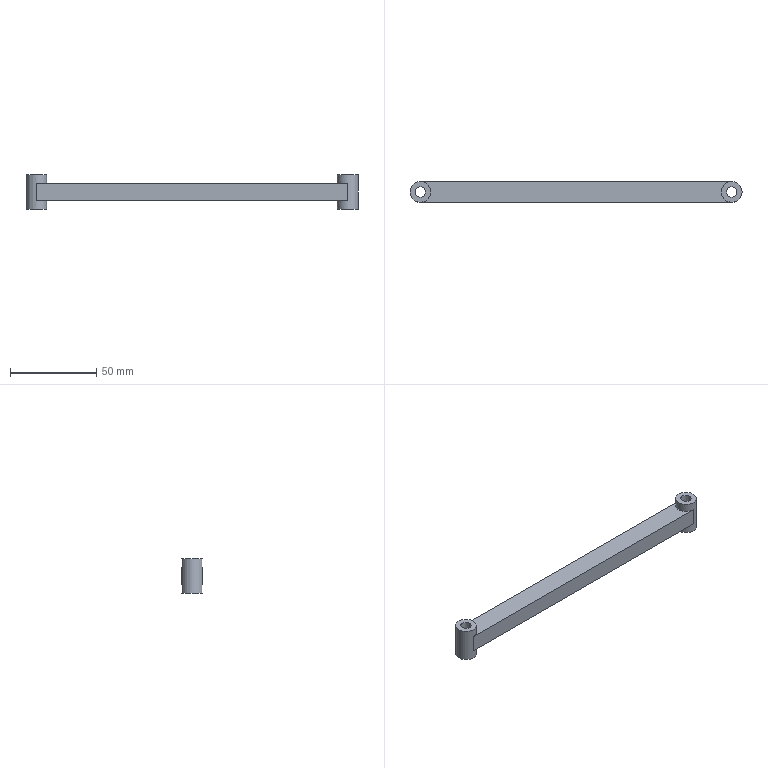Component | NX | CON_ROD2 | 1 solid | 12 faces | box 192 x 12 x 20 mm | volume 23862 mm3 | plane 8 | cylinder 4 | commonest cylinder face diameters 12 x2 6 x2
STEP:
#1=CARTESIAN_POINT('',(0.,0.,0.));
#2=DIRECTION('',(0.,0.,1.));
#3=DIRECTION('',(1.,0.,0.));
#4=AXIS2_PLACEMENT_3D('',#1,#2,#3);
#5=CARTESIAN_POINT('',(6.,65.,16.));
#6=VERTEX_POINT('',#5);
#7=CARTESIAN_POINT('',(-0.,65.,16.));
#8=DIRECTION('',(0.,0.,1.));
#9=DIRECTION('',(1.,0.,0.));
#10=AXIS2_PLACEMENT_3D('',#7,#8,#9);
#11=CIRCLE('',#10,6.);
#12=CARTESIAN_POINT('',(-0.,65.,36.));
#13=DIRECTION('',(0.,0.,-1.));
#14=DIRECTION('',(-1.,0.,0.));
#15=AXIS2_PLACEMENT_3D('',#12,#13,#14);
#16=CYLINDRICAL_SURFACE('',#15,6.);
#17=CARTESIAN_POINT('',(9.425,20.));
#18=DIRECTION('',(-1.,0.));
#19=VECTOR('',#18,1.);
#20=LINE('',#17,#19);
#21=(GEOMETRIC_REPRESENTATION_CONTEXT(2)PARAMETRIC_REPRESENTATION_CONTEXT()REPRESENTATION_CONTEXT('',''));
#22=DEFINITIONAL_REPRESENTATION('',(#20),#21);
#23=PCURVE('',#16,#22);
#24=CARTESIAN_POINT('',(-0.,65.,16.));
#25=DIRECTION('',(0.,0.,1.));
#26=DIRECTION('',(1.,0.,0.));
#27=AXIS2_PLACEMENT_3D('',#24,#25,#26);
#28=PLANE('',#27);
#29=CARTESIAN_POINT('',(0.,0.));
#30=DIRECTION('',(1.,0.));
#31=AXIS2_PLACEMENT_2D('',#29,#30);
#32=CIRCLE('',#31,6.);
#33=(GEOMETRIC_REPRESENTATION_CONTEXT(2)PARAMETRIC_REPRESENTATION_CONTEXT()REPRESENTATION_CONTEXT('',''));
#34=DEFINITIONAL_REPRESENTATION('',(#32),#33);
#35=PCURVE('',#28,#34);
#36=SURFACE_CURVE('',#11,(#23,#35),.PCURVE_S1.);
#37=EDGE_CURVE('',#6,#6,#36,.T.);
#38=ORIENTED_EDGE('',*,*,#37,.T.);
#39=CARTESIAN_POINT('',(6.,65.,21.));
#40=VERTEX_POINT('',#39);
#41=CARTESIAN_POINT('',(6.,65.,21.));
#42=CARTESIAN_POINT('',(6.,65.,16.));
#43=B_SPLINE_CURVE_WITH_KNOTS('',1,(#41,#42),.UNSPECIFIED.,.F.,.F.,(2,2),(15.,20.),.PIECEWISE_BEZIER_KNOTS.);
#44=CARTESIAN_POINT('',(3.142,0.));
#45=DIRECTION('',(0.,1.));
#46=VECTOR('',#45,1.);
#47=LINE('',#44,#46);
#48=(GEOMETRIC_REPRESENTATION_CONTEXT(2)PARAMETRIC_REPRESENTATION_CONTEXT()REPRESENTATION_CONTEXT('',''));
#49=DEFINITIONAL_REPRESENTATION('',(#47),#48);
#50=PCURVE('',#16,#49);
#51=CARTESIAN_POINT('',(9.425,0.));
#52=DIRECTION('',(0.,1.));
#53=VECTOR('',#52,1.);
#54=LINE('',#51,#53);
#55=(GEOMETRIC_REPRESENTATION_CONTEXT(2)PARAMETRIC_REPRESENTATION_CONTEXT()REPRESENTATION_CONTEXT('',''));
#56=DEFINITIONAL_REPRESENTATION('',(#54),#55);
#57=PCURVE('',#16,#56);
#58=SEAM_CURVE('',#43,(#50,#57),.PCURVE_S1.);
#59=EDGE_CURVE('',#40,#6,#58,.T.);
#60=ORIENTED_EDGE('',*,*,#59,.F.);
#61=CARTESIAN_POINT('',(-0.,59.,21.));
#62=VERTEX_POINT('',#61);
#63=CARTESIAN_POINT('',(-0.,65.,21.));
#64=DIRECTION('',(0.,0.,-1.));
#65=DIRECTION('',(-1.,0.,0.));
#66=AXIS2_PLACEMENT_3D('',#63,#64,#65);
#67=CIRCLE('',#66,6.);
#68=CARTESIAN_POINT('',(0.,15.));
#69=DIRECTION('',(1.,0.));
#70=VECTOR('',#69,1.);
#71=LINE('',#68,#70);
#72=(GEOMETRIC_REPRESENTATION_CONTEXT(2)PARAMETRIC_REPRESENTATION_CONTEXT()REPRESENTATION_CONTEXT('',''));
#73=DEFINITIONAL_REPRESENTATION('',(#71),#72);
#74=PCURVE('',#16,#73);
#75=CARTESIAN_POINT('',(-0.,65.,21.));
#76=DIRECTION('',(0.,0.,-1.));
#77=DIRECTION('',(1.,0.,0.));
#78=AXIS2_PLACEMENT_3D('',#75,#76,#77);
#79=PLANE('',#78);
#80=CARTESIAN_POINT('',(0.,0.));
#81=DIRECTION('',(-1.,0.));
#82=AXIS2_PLACEMENT_2D('',#80,#81);
#83=CIRCLE('',#82,6.);
#84=(GEOMETRIC_REPRESENTATION_CONTEXT(2)PARAMETRIC_REPRESENTATION_CONTEXT()REPRESENTATION_CONTEXT('',''));
#85=DEFINITIONAL_REPRESENTATION('',(#83),#84);
#86=PCURVE('',#79,#85);
#87=SURFACE_CURVE('',#67,(#74,#86),.PCURVE_S1.);
#88=EDGE_CURVE('',#40,#62,#87,.T.);
#89=ORIENTED_EDGE('',*,*,#88,.T.);
#90=CARTESIAN_POINT('',(-0.,59.,31.));
#91=VERTEX_POINT('',#90);
#92=CARTESIAN_POINT('',(-0.,59.,21.));
#93=DIRECTION('',(0.,0.,1.));
#94=VECTOR('',#93,1.);
#95=LINE('',#92,#94);
#96=CARTESIAN_POINT('',(4.712,15.));
#97=DIRECTION('',(0.,-1.));
#98=VECTOR('',#97,1.);
#99=LINE('',#96,#98);
#100=(GEOMETRIC_REPRESENTATION_CONTEXT(2)PARAMETRIC_REPRESENTATION_CONTEXT()REPRESENTATION_CONTEXT('',''));
#101=DEFINITIONAL_REPRESENTATION('',(#99),#100);
#102=PCURVE('',#16,#101);
#103=CARTESIAN_POINT('',(-0.,59.,21.));
#104=DIRECTION('',(0.,-1.,0.));
#105=DIRECTION('',(0.,0.,-1.));
#106=AXIS2_PLACEMENT_3D('',#103,#104,#105);
#107=PLANE('',#106);
#108=CARTESIAN_POINT('',(0.,0.));
#109=DIRECTION('',(-1.,0.));
#110=VECTOR('',#109,1.);
#111=LINE('',#108,#110);
#112=(GEOMETRIC_REPRESENTATION_CONTEXT(2)PARAMETRIC_REPRESENTATION_CONTEXT()REPRESENTATION_CONTEXT('',''));
#113=DEFINITIONAL_REPRESENTATION('',(#111),#112);
#114=PCURVE('',#107,#113);
#115=SURFACE_CURVE('',#95,(#102,#114),.PCURVE_S1.);
#116=EDGE_CURVE('',#62,#91,#115,.T.);
#117=ORIENTED_EDGE('',*,*,#116,.T.);
#118=CARTESIAN_POINT('',(6.,65.,31.));
#119=VERTEX_POINT('',#118);
#120=CARTESIAN_POINT('',(-0.,65.,31.));
#121=DIRECTION('',(0.,0.,1.));
#122=DIRECTION('',(-1.,0.,0.));
#123=AXIS2_PLACEMENT_3D('',#120,#121,#122);
#124=CIRCLE('',#123,6.);
#125=CARTESIAN_POINT('',(6.283,5.));
#126=DIRECTION('',(-1.,0.));
#127=VECTOR('',#126,1.);
#128=LINE('',#125,#127);
#129=(GEOMETRIC_REPRESENTATION_CONTEXT(2)PARAMETRIC_REPRESENTATION_CONTEXT()REPRESENTATION_CONTEXT('',''));
#130=DEFINITIONAL_REPRESENTATION('',(#128),#129);
#131=PCURVE('',#16,#130);
#132=CARTESIAN_POINT('',(-0.,65.,31.));
#133=DIRECTION('',(0.,0.,-1.));
#134=DIRECTION('',(1.,0.,0.));
#135=AXIS2_PLACEMENT_3D('',#132,#133,#134);
#136=PLANE('',#135);
#137=CARTESIAN_POINT('',(-6.,0.));
#138=CARTESIAN_POINT('',(-6.,10.392));
#139=CARTESIAN_POINT('',(3.,5.196));
#140=CARTESIAN_POINT('',(12.,0.));
#141=CARTESIAN_POINT('',(3.,-5.196));
#142=CARTESIAN_POINT('',(-6.,-10.392));
#143=CARTESIAN_POINT('',(-6.,0.));
#144=(BOUNDED_CURVE()B_SPLINE_CURVE(2,(#137,#138,#139,#140,#141,#142,#143),.UNSPECIFIED.,.T.,.F.)B_SPLINE_CURVE_WITH_KNOTS((1,2,2,2,2,1),(-2.094,0.,2.094,4.189,6.283,8.378),.UNSPECIFIED.)CURVE()GEOMETRIC_REPRESENTATION_ITEM()RATIONAL_B_SPLINE_CURVE((1.,0.5,1.,0.5,1.,0.5,1.))REPRESENTATION_ITEM(''));
#145=(GEOMETRIC_REPRESENTATION_CONTEXT(2)PARAMETRIC_REPRESENTATION_CONTEXT()REPRESENTATION_CONTEXT('',''));
#146=DEFINITIONAL_REPRESENTATION('',(#144),#145);
#147=PCURVE('',#136,#146);
#148=SURFACE_CURVE('',#124,(#131,#147),.PCURVE_S1.);
#149=EDGE_CURVE('',#91,#119,#148,.T.);
#150=ORIENTED_EDGE('',*,*,#149,.T.);
#151=CARTESIAN_POINT('',(6.,65.,36.));
#152=VERTEX_POINT('',#151);
#153=CARTESIAN_POINT('',(6.,65.,36.));
#154=CARTESIAN_POINT('',(6.,65.,31.));
#155=B_SPLINE_CURVE_WITH_KNOTS('',1,(#153,#154),.UNSPECIFIED.,.F.,.F.,(2,2),(0.,5.),.PIECEWISE_BEZIER_KNOTS.);
#156=CARTESIAN_POINT('',(3.142,0.));
#157=DIRECTION('',(0.,1.));
#158=VECTOR('',#157,1.);
#159=LINE('',#156,#158);
#160=(GEOMETRIC_REPRESENTATION_CONTEXT(2)PARAMETRIC_REPRESENTATION_CONTEXT()REPRESENTATION_CONTEXT('',''));
#161=DEFINITIONAL_REPRESENTATION('',(#159),#160);
#162=PCURVE('',#16,#161);
#163=CARTESIAN_POINT('',(9.425,0.));
#164=DIRECTION('',(0.,1.));
#165=VECTOR('',#164,1.);
#166=LINE('',#163,#165);
#167=(GEOMETRIC_REPRESENTATION_CONTEXT(2)PARAMETRIC_REPRESENTATION_CONTEXT()REPRESENTATION_CONTEXT('',''));
#168=DEFINITIONAL_REPRESENTATION('',(#166),#167);
#169=PCURVE('',#16,#168);
#170=SEAM_CURVE('',#155,(#162,#169),.PCURVE_S1.);
#171=EDGE_CURVE('',#152,#119,#170,.T.);
#172=ORIENTED_EDGE('',*,*,#171,.F.);
#173=CARTESIAN_POINT('',(-0.,65.,36.));
#174=DIRECTION('',(0.,0.,1.));
#175=DIRECTION('',(1.,0.,0.));
#176=AXIS2_PLACEMENT_3D('',#173,#174,#175);
#177=CIRCLE('',#176,6.);
#178=CARTESIAN_POINT('',(9.425,0.));
#179=DIRECTION('',(-1.,0.));
#180=VECTOR('',#179,1.);
#181=LINE('',#178,#180);
#182=(GEOMETRIC_REPRESENTATION_CONTEXT(2)PARAMETRIC_REPRESENTATION_CONTEXT()REPRESENTATION_CONTEXT('',''));
#183=DEFINITIONAL_REPRESENTATION('',(#181),#182);
#184=PCURVE('',#16,#183);
#185=CARTESIAN_POINT('',(-0.,65.,36.));
#186=DIRECTION('',(0.,0.,1.));
#187=DIRECTION('',(1.,0.,0.));
#188=AXIS2_PLACEMENT_3D('',#185,#186,#187);
#189=PLANE('',#188);
#190=CARTESIAN_POINT('',(0.,0.));
#191=DIRECTION('',(1.,0.));
#192=AXIS2_PLACEMENT_2D('',#190,#191);
#193=CIRCLE('',#192,6.);
#194=(GEOMETRIC_REPRESENTATION_CONTEXT(2)PARAMETRIC_REPRESENTATION_CONTEXT()REPRESENTATION_CONTEXT('',''));
#195=DEFINITIONAL_REPRESENTATION('',(#193),#194);
#196=PCURVE('',#189,#195);
#197=SURFACE_CURVE('',#177,(#184,#196),.PCURVE_S1.);
#198=EDGE_CURVE('',#152,#152,#197,.T.);
#199=ORIENTED_EDGE('',*,*,#198,.F.);
#200=ORIENTED_EDGE('',*,*,#171,.T.);
#201=CARTESIAN_POINT('',(-0.,71.,31.));
#202=VERTEX_POINT('',#201);
#203=CARTESIAN_POINT('',(-0.,65.,31.));
#204=DIRECTION('',(0.,0.,1.));
#205=DIRECTION('',(-1.,0.,0.));
#206=AXIS2_PLACEMENT_3D('',#203,#204,#205);
#207=CIRCLE('',#206,6.);
#208=CARTESIAN_POINT('',(12.566,5.));
#209=DIRECTION('',(-1.,0.));
#210=VECTOR('',#209,1.);
#211=LINE('',#208,#210);
#212=(GEOMETRIC_REPRESENTATION_CONTEXT(2)PARAMETRIC_REPRESENTATION_CONTEXT()REPRESENTATION_CONTEXT('',''));
#213=DEFINITIONAL_REPRESENTATION('',(#211),#212);
#214=PCURVE('',#16,#213);
#215=CARTESIAN_POINT('',(-6.,0.));
#216=CARTESIAN_POINT('',(-6.,10.392));
#217=CARTESIAN_POINT('',(3.,5.196));
#218=CARTESIAN_POINT('',(12.,0.));
#219=CARTESIAN_POINT('',(3.,-5.196));
#220=CARTESIAN_POINT('',(-6.,-10.392));
#221=CARTESIAN_POINT('',(-6.,0.));
#222=(BOUNDED_CURVE()B_SPLINE_CURVE(2,(#215,#216,#217,#218,#219,#220,#221),.UNSPECIFIED.,.T.,.F.)B_SPLINE_CURVE_WITH_KNOTS((1,2,2,2,2,1),(-2.094,0.,2.094,4.189,6.283,8.378),.UNSPECIFIED.)CURVE()GEOMETRIC_REPRESENTATION_ITEM()RATIONAL_B_SPLINE_CURVE((1.,0.5,1.,0.5,1.,0.5,1.))REPRESENTATION_ITEM(''));
#223=(GEOMETRIC_REPRESENTATION_CONTEXT(2)PARAMETRIC_REPRESENTATION_CONTEXT()REPRESENTATION_CONTEXT('',''));
#224=DEFINITIONAL_REPRESENTATION('',(#222),#223);
#225=PCURVE('',#136,#224);
#226=SURFACE_CURVE('',#207,(#214,#225),.PCURVE_S1.);
#227=EDGE_CURVE('',#119,#202,#226,.T.);
#228=ORIENTED_EDGE('',*,*,#227,.T.);
#229=CARTESIAN_POINT('',(-0.,71.,21.));
#230=VERTEX_POINT('',#229);
#231=CARTESIAN_POINT('',(-0.,71.,21.));
#232=DIRECTION('',(0.,0.,1.));
#233=VECTOR('',#232,1.);
#234=LINE('',#231,#233);
#235=CARTESIAN_POINT('',(7.854,15.));
#236=DIRECTION('',(0.,-1.));
#237=VECTOR('',#236,1.);
#238=LINE('',#235,#237);
#239=(GEOMETRIC_REPRESENTATION_CONTEXT(2)PARAMETRIC_REPRESENTATION_CONTEXT()REPRESENTATION_CONTEXT('',''));
#240=DEFINITIONAL_REPRESENTATION('',(#238),#239);
#241=PCURVE('',#16,#240);
#242=CARTESIAN_POINT('',(-0.,71.,21.));
#243=DIRECTION('',(0.,-1.,0.));
#244=DIRECTION('',(0.,0.,-1.));
#245=AXIS2_PLACEMENT_3D('',#242,#243,#244);
#246=PLANE('',#245);
#247=CARTESIAN_POINT('',(0.,0.));
#248=DIRECTION('',(-1.,0.));
#249=VECTOR('',#248,1.);
#250=LINE('',#247,#249);
#251=(GEOMETRIC_REPRESENTATION_CONTEXT(2)PARAMETRIC_REPRESENTATION_CONTEXT()REPRESENTATION_CONTEXT('',''));
#252=DEFINITIONAL_REPRESENTATION('',(#250),#251);
#253=PCURVE('',#246,#252);
#254=SURFACE_CURVE('',#234,(#241,#253),.PCURVE_S1.);
#255=EDGE_CURVE('',#230,#202,#254,.T.);
#256=ORIENTED_EDGE('',*,*,#255,.F.);
#257=CARTESIAN_POINT('',(-0.,65.,21.));
#258=DIRECTION('',(0.,0.,-1.));
#259=DIRECTION('',(-1.,0.,0.));
#260=AXIS2_PLACEMENT_3D('',#257,#258,#259);
#261=CIRCLE('',#260,6.);
#262=CARTESIAN_POINT('',(6.283,15.));
#263=DIRECTION('',(1.,0.));
#264=VECTOR('',#263,1.);
#265=LINE('',#262,#264);
#266=(GEOMETRIC_REPRESENTATION_CONTEXT(2)PARAMETRIC_REPRESENTATION_CONTEXT()REPRESENTATION_CONTEXT('',''));
#267=DEFINITIONAL_REPRESENTATION('',(#265),#266);
#268=PCURVE('',#16,#267);
#269=CARTESIAN_POINT('',(0.,0.));
#270=DIRECTION('',(-1.,0.));
#271=AXIS2_PLACEMENT_2D('',#269,#270);
#272=CIRCLE('',#271,6.);
#273=(GEOMETRIC_REPRESENTATION_CONTEXT(2)PARAMETRIC_REPRESENTATION_CONTEXT()REPRESENTATION_CONTEXT('',''));
#274=DEFINITIONAL_REPRESENTATION('',(#272),#273);
#275=PCURVE('',#79,#274);
#276=SURFACE_CURVE('',#261,(#268,#275),.PCURVE_S1.);
#277=EDGE_CURVE('',#230,#40,#276,.T.);
#278=ORIENTED_EDGE('',*,*,#277,.T.);
#279=ORIENTED_EDGE('',*,*,#59,.T.);
#280=EDGE_LOOP('',(#38,#60,#89,#117,#150,#172,#199,#200,#228,#256,#278,#279));
#281=FACE_BOUND('',#280,.T.);
#282=ADVANCED_FACE('',(#281),#16,.T.);
#283=CARTESIAN_POINT('',(-3.,65.,36.));
#284=VERTEX_POINT('',#283);
#285=CARTESIAN_POINT('',(-0.,65.,36.));
#286=DIRECTION('',(0.,0.,-1.));
#287=DIRECTION('',(-1.,0.,0.));
#288=AXIS2_PLACEMENT_3D('',#285,#286,#287);
#289=CIRCLE('',#288,3.);
#290=CARTESIAN_POINT('',(-3.,0.));
#291=CARTESIAN_POINT('',(-3.,5.196));
#292=CARTESIAN_POINT('',(1.5,2.598));
#293=CARTESIAN_POINT('',(6.,0.));
#294=CARTESIAN_POINT('',(1.5,-2.598));
#295=CARTESIAN_POINT('',(-3.,-5.196));
#296=CARTESIAN_POINT('',(-3.,0.));
#297=(BOUNDED_CURVE()B_SPLINE_CURVE(2,(#290,#291,#292,#293,#294,#295,#296),.UNSPECIFIED.,.T.,.F.)B_SPLINE_CURVE_WITH_KNOTS((1,2,2,2,2,1),(-2.094,0.,2.094,4.189,6.283,8.378),.UNSPECIFIED.)CURVE()GEOMETRIC_REPRESENTATION_ITEM()RATIONAL_B_SPLINE_CURVE((1.,0.5,1.,0.5,1.,0.5,1.))REPRESENTATION_ITEM(''));
#298=(GEOMETRIC_REPRESENTATION_CONTEXT(2)PARAMETRIC_REPRESENTATION_CONTEXT()REPRESENTATION_CONTEXT('',''));
#299=DEFINITIONAL_REPRESENTATION('',(#297),#298);
#300=PCURVE('',#189,#299);
#301=CARTESIAN_POINT('',(-0.,65.,36.));
#302=DIRECTION('',(0.,0.,-1.));
#303=DIRECTION('',(-1.,0.,0.));
#304=AXIS2_PLACEMENT_3D('',#301,#302,#303);
#305=CYLINDRICAL_SURFACE('',#304,3.);
#306=CARTESIAN_POINT('',(0.,0.));
#307=DIRECTION('',(1.,0.));
#308=VECTOR('',#307,1.);
#309=LINE('',#306,#308);
#310=(GEOMETRIC_REPRESENTATION_CONTEXT(2)PARAMETRIC_REPRESENTATION_CONTEXT()REPRESENTATION_CONTEXT('',''));
#311=DEFINITIONAL_REPRESENTATION('',(#309),#310);
#312=PCURVE('',#305,#311);
#313=SURFACE_CURVE('',#289,(#300,#312),.PCURVE_S1.);
#314=EDGE_CURVE('',#284,#284,#313,.T.);
#315=ORIENTED_EDGE('',*,*,#314,.T.);
#316=EDGE_LOOP('',(#315));
#317=FACE_BOUND('',#316,.T.);
#318=ORIENTED_EDGE('',*,*,#198,.T.);
#319=EDGE_LOOP('',(#318));
#320=FACE_BOUND('',#319,.T.);
#321=ADVANCED_FACE('',(#317,#320),#189,.T.);
#322=CARTESIAN_POINT('',(3.,65.,16.));
#323=VERTEX_POINT('',#322);
#324=CARTESIAN_POINT('',(-3.,65.,16.));
#325=VERTEX_POINT('',#324);
#326=CARTESIAN_POINT('',(-0.,65.,16.));
#327=DIRECTION('',(0.,0.,1.));
#328=DIRECTION('',(1.,0.,0.));
#329=AXIS2_PLACEMENT_3D('',#326,#327,#328);
#330=CIRCLE('',#329,3.);
#331=CARTESIAN_POINT('',(0.,0.));
#332=DIRECTION('',(1.,0.));
#333=AXIS2_PLACEMENT_2D('',#331,#332);
#334=CIRCLE('',#333,3.);
#335=(GEOMETRIC_REPRESENTATION_CONTEXT(2)PARAMETRIC_REPRESENTATION_CONTEXT()REPRESENTATION_CONTEXT('',''));
#336=DEFINITIONAL_REPRESENTATION('',(#334),#335);
#337=PCURVE('',#28,#336);
#338=CARTESIAN_POINT('',(3.142,20.));
#339=DIRECTION('',(-1.,0.));
#340=VECTOR('',#339,1.);
#341=LINE('',#338,#340);
#342=(GEOMETRIC_REPRESENTATION_CONTEXT(2)PARAMETRIC_REPRESENTATION_CONTEXT()REPRESENTATION_CONTEXT('',''));
#343=DEFINITIONAL_REPRESENTATION('',(#341),#342);
#344=PCURVE('',#305,#343);
#345=SURFACE_CURVE('',#330,(#337,#344),.PCURVE_S1.);
#346=EDGE_CURVE('',#323,#325,#345,.T.);
#347=ORIENTED_EDGE('',*,*,#346,.T.);
#348=CARTESIAN_POINT('',(-0.,65.,16.));
#349=DIRECTION('',(0.,0.,1.));
#350=DIRECTION('',(1.,0.,0.));
#351=AXIS2_PLACEMENT_3D('',#348,#349,#350);
#352=CIRCLE('',#351,3.);
#353=CARTESIAN_POINT('',(0.,0.));
#354=DIRECTION('',(1.,0.));
#355=AXIS2_PLACEMENT_2D('',#353,#354);
#356=CIRCLE('',#355,3.);
#357=(GEOMETRIC_REPRESENTATION_CONTEXT(2)PARAMETRIC_REPRESENTATION_CONTEXT()REPRESENTATION_CONTEXT('',''));
#358=DEFINITIONAL_REPRESENTATION('',(#356),#357);
#359=PCURVE('',#28,#358);
#360=CARTESIAN_POINT('',(9.425,20.));
#361=DIRECTION('',(-1.,0.));
#362=VECTOR('',#361,1.);
#363=LINE('',#360,#362);
#364=(GEOMETRIC_REPRESENTATION_CONTEXT(2)PARAMETRIC_REPRESENTATION_CONTEXT()REPRESENTATION_CONTEXT('',''));
#365=DEFINITIONAL_REPRESENTATION('',(#363),#364);
#366=PCURVE('',#305,#365);
#367=SURFACE_CURVE('',#352,(#359,#366),.PCURVE_S1.);
#368=EDGE_CURVE('',#325,#323,#367,.T.);
#369=ORIENTED_EDGE('',*,*,#368,.T.);
#370=EDGE_LOOP('',(#347,#369));
#371=FACE_BOUND('',#370,.T.);
#372=ORIENTED_EDGE('',*,*,#37,.F.);
#373=EDGE_LOOP('',(#372));
#374=FACE_BOUND('',#373,.T.);
#375=ADVANCED_FACE('',(#371,#374),#28,.F.);
#376=CARTESIAN_POINT('',(186.,65.,36.));
#377=VERTEX_POINT('',#376);
#378=CARTESIAN_POINT('',(180.,65.,36.));
#379=DIRECTION('',(0.,0.,1.));
#380=DIRECTION('',(1.,0.,0.));
#381=AXIS2_PLACEMENT_3D('',#378,#379,#380);
#382=CIRCLE('',#381,6.);
#383=CARTESIAN_POINT('',(180.,65.,36.));
#384=DIRECTION('',(0.,0.,-1.));
#385=DIRECTION('',(-1.,0.,0.));
#386=AXIS2_PLACEMENT_3D('',#383,#384,#385);
#387=CYLINDRICAL_SURFACE('',#386,6.);
#388=CARTESIAN_POINT('',(9.425,0.));
#389=DIRECTION('',(-1.,0.));
#390=VECTOR('',#389,1.);
#391=LINE('',#388,#390);
#392=(GEOMETRIC_REPRESENTATION_CONTEXT(2)PARAMETRIC_REPRESENTATION_CONTEXT()REPRESENTATION_CONTEXT('',''));
#393=DEFINITIONAL_REPRESENTATION('',(#391),#392);
#394=PCURVE('',#387,#393);
#395=CARTESIAN_POINT('',(180.,65.,36.));
#396=DIRECTION('',(0.,0.,1.));
#397=DIRECTION('',(1.,0.,0.));
#398=AXIS2_PLACEMENT_3D('',#395,#396,#397);
#399=PLANE('',#398);
#400=CARTESIAN_POINT('',(0.,0.));
#401=DIRECTION('',(1.,0.));
#402=AXIS2_PLACEMENT_2D('',#400,#401);
#403=CIRCLE('',#402,6.);
#404=(GEOMETRIC_REPRESENTATION_CONTEXT(2)PARAMETRIC_REPRESENTATION_CONTEXT()REPRESENTATION_CONTEXT('',''));
#405=DEFINITIONAL_REPRESENTATION('',(#403),#404);
#406=PCURVE('',#399,#405);
#407=SURFACE_CURVE('',#382,(#394,#406),.PCURVE_S1.);
#408=EDGE_CURVE('',#377,#377,#407,.T.);
#409=ORIENTED_EDGE('',*,*,#408,.F.);
#410=CARTESIAN_POINT('',(186.,65.,16.));
#411=VERTEX_POINT('',#410);
#412=CARTESIAN_POINT('',(186.,65.,36.));
#413=CARTESIAN_POINT('',(186.,65.,16.));
#414=B_SPLINE_CURVE_WITH_KNOTS('',1,(#412,#413),.UNSPECIFIED.,.F.,.F.,(2,2),(0.,20.),.PIECEWISE_BEZIER_KNOTS.);
#415=CARTESIAN_POINT('',(9.425,0.));
#416=DIRECTION('',(0.,1.));
#417=VECTOR('',#416,1.);
#418=LINE('',#415,#417);
#419=(GEOMETRIC_REPRESENTATION_CONTEXT(2)PARAMETRIC_REPRESENTATION_CONTEXT()REPRESENTATION_CONTEXT('',''));
#420=DEFINITIONAL_REPRESENTATION('',(#418),#419);
#421=PCURVE('',#387,#420);
#422=CARTESIAN_POINT('',(3.142,0.));
#423=DIRECTION('',(0.,1.));
#424=VECTOR('',#423,1.);
#425=LINE('',#422,#424);
#426=(GEOMETRIC_REPRESENTATION_CONTEXT(2)PARAMETRIC_REPRESENTATION_CONTEXT()REPRESENTATION_CONTEXT('',''));
#427=DEFINITIONAL_REPRESENTATION('',(#425),#426);
#428=PCURVE('',#387,#427);
#429=SEAM_CURVE('',#414,(#421,#428),.PCURVE_S1.);
#430=EDGE_CURVE('',#377,#411,#429,.T.);
#431=ORIENTED_EDGE('',*,*,#430,.T.);
#432=CARTESIAN_POINT('',(180.,65.,16.));
#433=DIRECTION('',(0.,0.,1.));
#434=DIRECTION('',(1.,0.,0.));
#435=AXIS2_PLACEMENT_3D('',#432,#433,#434);
#436=CIRCLE('',#435,6.);
#437=CARTESIAN_POINT('',(9.425,20.));
#438=DIRECTION('',(-1.,0.));
#439=VECTOR('',#438,1.);
#440=LINE('',#437,#439);
#441=(GEOMETRIC_REPRESENTATION_CONTEXT(2)PARAMETRIC_REPRESENTATION_CONTEXT()REPRESENTATION_CONTEXT('',''));
#442=DEFINITIONAL_REPRESENTATION('',(#440),#441);
#443=PCURVE('',#387,#442);
#444=CARTESIAN_POINT('',(180.,65.,16.));
#445=DIRECTION('',(0.,0.,1.));
#446=DIRECTION('',(1.,0.,0.));
#447=AXIS2_PLACEMENT_3D('',#444,#445,#446);
#448=PLANE('',#447);
#449=CARTESIAN_POINT('',(0.,0.));
#450=DIRECTION('',(1.,0.));
#451=AXIS2_PLACEMENT_2D('',#449,#450);
#452=CIRCLE('',#451,6.);
#453=(GEOMETRIC_REPRESENTATION_CONTEXT(2)PARAMETRIC_REPRESENTATION_CONTEXT()REPRESENTATION_CONTEXT('',''));
#454=DEFINITIONAL_REPRESENTATION('',(#452),#453);
#455=PCURVE('',#448,#454);
#456=SURFACE_CURVE('',#436,(#443,#455),.PCURVE_S1.);
#457=EDGE_CURVE('',#411,#411,#456,.T.);
#458=ORIENTED_EDGE('',*,*,#457,.T.);
#459=ORIENTED_EDGE('',*,*,#430,.F.);
#460=EDGE_LOOP('',(#409,#431,#458,#459));
#461=FACE_BOUND('',#460,.T.);
#462=CARTESIAN_POINT('',(180.,59.,21.));
#463=VERTEX_POINT('',#462);
#464=CARTESIAN_POINT('',(180.,59.,31.));
#465=VERTEX_POINT('',#464);
#466=CARTESIAN_POINT('',(180.,59.,21.));
#467=DIRECTION('',(0.,0.,1.));
#468=VECTOR('',#467,1.);
#469=LINE('',#466,#468);
#470=CARTESIAN_POINT('',(4.712,15.));
#471=DIRECTION('',(0.,-1.));
#472=VECTOR('',#471,1.);
#473=LINE('',#470,#472);
#474=(GEOMETRIC_REPRESENTATION_CONTEXT(2)PARAMETRIC_REPRESENTATION_CONTEXT()REPRESENTATION_CONTEXT('',''));
#475=DEFINITIONAL_REPRESENTATION('',(#473),#474);
#476=PCURVE('',#387,#475);
#477=CARTESIAN_POINT('',(0.,180.));
#478=DIRECTION('',(-1.,0.));
#479=VECTOR('',#478,1.);
#480=LINE('',#477,#479);
#481=(GEOMETRIC_REPRESENTATION_CONTEXT(2)PARAMETRIC_REPRESENTATION_CONTEXT()REPRESENTATION_CONTEXT('',''));
#482=DEFINITIONAL_REPRESENTATION('',(#480),#481);
#483=PCURVE('',#107,#482);
#484=SURFACE_CURVE('',#469,(#476,#483),.PCURVE_S1.);
#485=EDGE_CURVE('',#463,#465,#484,.T.);
#486=ORIENTED_EDGE('',*,*,#485,.F.);
#487=CARTESIAN_POINT('',(180.,71.,21.));
#488=VERTEX_POINT('',#487);
#489=CARTESIAN_POINT('',(180.,65.,21.));
#490=DIRECTION('',(0.,0.,-1.));
#491=DIRECTION('',(-1.,0.,0.));
#492=AXIS2_PLACEMENT_3D('',#489,#490,#491);
#493=CIRCLE('',#492,6.);
#494=CARTESIAN_POINT('',(0.,15.));
#495=DIRECTION('',(1.,0.));
#496=VECTOR('',#495,1.);
#497=LINE('',#494,#496);
#498=(GEOMETRIC_REPRESENTATION_CONTEXT(2)PARAMETRIC_REPRESENTATION_CONTEXT()REPRESENTATION_CONTEXT('',''));
#499=DEFINITIONAL_REPRESENTATION('',(#497),#498);
#500=PCURVE('',#387,#499);
#501=CARTESIAN_POINT('',(180.,0.));
#502=DIRECTION('',(-1.,0.));
#503=AXIS2_PLACEMENT_2D('',#501,#502);
#504=CIRCLE('',#503,6.);
#505=(GEOMETRIC_REPRESENTATION_CONTEXT(2)PARAMETRIC_REPRESENTATION_CONTEXT()REPRESENTATION_CONTEXT('',''));
#506=DEFINITIONAL_REPRESENTATION('',(#504),#505);
#507=PCURVE('',#79,#506);
#508=SURFACE_CURVE('',#493,(#500,#507),.PCURVE_S1.);
#509=EDGE_CURVE('',#463,#488,#508,.T.);
#510=ORIENTED_EDGE('',*,*,#509,.T.);
#511=CARTESIAN_POINT('',(180.,71.,31.));
#512=VERTEX_POINT('',#511);
#513=CARTESIAN_POINT('',(180.,71.,21.));
#514=DIRECTION('',(0.,0.,1.));
#515=VECTOR('',#514,1.);
#516=LINE('',#513,#515);
#517=CARTESIAN_POINT('',(7.854,15.));
#518=DIRECTION('',(0.,-1.));
#519=VECTOR('',#518,1.);
#520=LINE('',#517,#519);
#521=(GEOMETRIC_REPRESENTATION_CONTEXT(2)PARAMETRIC_REPRESENTATION_CONTEXT()REPRESENTATION_CONTEXT('',''));
#522=DEFINITIONAL_REPRESENTATION('',(#520),#521);
#523=PCURVE('',#387,#522);
#524=CARTESIAN_POINT('',(0.,180.));
#525=DIRECTION('',(-1.,0.));
#526=VECTOR('',#525,1.);
#527=LINE('',#524,#526);
#528=(GEOMETRIC_REPRESENTATION_CONTEXT(2)PARAMETRIC_REPRESENTATION_CONTEXT()REPRESENTATION_CONTEXT('',''));
#529=DEFINITIONAL_REPRESENTATION('',(#527),#528);
#530=PCURVE('',#246,#529);
#531=SURFACE_CURVE('',#516,(#523,#530),.PCURVE_S1.);
#532=EDGE_CURVE('',#488,#512,#531,.T.);
#533=ORIENTED_EDGE('',*,*,#532,.T.);
#534=CARTESIAN_POINT('',(180.,65.,31.));
#535=DIRECTION('',(0.,0.,1.));
#536=DIRECTION('',(-1.,0.,0.));
#537=AXIS2_PLACEMENT_3D('',#534,#535,#536);
#538=CIRCLE('',#537,6.);
#539=CARTESIAN_POINT('',(12.566,5.));
#540=DIRECTION('',(-1.,0.));
#541=VECTOR('',#540,1.);
#542=LINE('',#539,#541);
#543=(GEOMETRIC_REPRESENTATION_CONTEXT(2)PARAMETRIC_REPRESENTATION_CONTEXT()REPRESENTATION_CONTEXT('',''));
#544=DEFINITIONAL_REPRESENTATION('',(#542),#543);
#545=PCURVE('',#387,#544);
#546=CARTESIAN_POINT('',(174.,0.));
#547=CARTESIAN_POINT('',(174.,10.392));
#548=CARTESIAN_POINT('',(183.,5.196));
#549=CARTESIAN_POINT('',(192.,0.));
#550=CARTESIAN_POINT('',(183.,-5.196));
#551=CARTESIAN_POINT('',(174.,-10.392));
#552=CARTESIAN_POINT('',(174.,0.));
#553=(BOUNDED_CURVE()B_SPLINE_CURVE(2,(#546,#547,#548,#549,#550,#551,#552),.UNSPECIFIED.,.T.,.F.)B_SPLINE_CURVE_WITH_KNOTS((1,2,2,2,2,1),(-2.094,0.,2.094,4.189,6.283,8.378),.UNSPECIFIED.)CURVE()GEOMETRIC_REPRESENTATION_ITEM()RATIONAL_B_SPLINE_CURVE((1.,0.5,1.,0.5,1.,0.5,1.))REPRESENTATION_ITEM(''));
#554=(GEOMETRIC_REPRESENTATION_CONTEXT(2)PARAMETRIC_REPRESENTATION_CONTEXT()REPRESENTATION_CONTEXT('',''));
#555=DEFINITIONAL_REPRESENTATION('',(#553),#554);
#556=PCURVE('',#136,#555);
#557=SURFACE_CURVE('',#538,(#545,#556),.PCURVE_S1.);
#558=EDGE_CURVE('',#512,#465,#557,.T.);
#559=ORIENTED_EDGE('',*,*,#558,.T.);
#560=EDGE_LOOP('',(#486,#510,#533,#559));
#561=FACE_BOUND('',#560,.T.);
#562=ADVANCED_FACE('',(#461,#561),#387,.T.);
#563=CARTESIAN_POINT('',(177.,65.,36.));
#564=VERTEX_POINT('',#563);
#565=CARTESIAN_POINT('',(180.,65.,36.));
#566=DIRECTION('',(0.,0.,-1.));
#567=DIRECTION('',(-1.,0.,0.));
#568=AXIS2_PLACEMENT_3D('',#565,#566,#567);
#569=CIRCLE('',#568,3.);
#570=CARTESIAN_POINT('',(-3.,0.));
#571=CARTESIAN_POINT('',(-3.,5.196));
#572=CARTESIAN_POINT('',(1.5,2.598));
#573=CARTESIAN_POINT('',(6.,0.));
#574=CARTESIAN_POINT('',(1.5,-2.598));
#575=CARTESIAN_POINT('',(-3.,-5.196));
#576=CARTESIAN_POINT('',(-3.,0.));
#577=(BOUNDED_CURVE()B_SPLINE_CURVE(2,(#570,#571,#572,#573,#574,#575,#576),.UNSPECIFIED.,.T.,.F.)B_SPLINE_CURVE_WITH_KNOTS((1,2,2,2,2,1),(-2.094,0.,2.094,4.189,6.283,8.378),.UNSPECIFIED.)CURVE()GEOMETRIC_REPRESENTATION_ITEM()RATIONAL_B_SPLINE_CURVE((1.,0.5,1.,0.5,1.,0.5,1.))REPRESENTATION_ITEM(''));
#578=(GEOMETRIC_REPRESENTATION_CONTEXT(2)PARAMETRIC_REPRESENTATION_CONTEXT()REPRESENTATION_CONTEXT('',''));
#579=DEFINITIONAL_REPRESENTATION('',(#577),#578);
#580=PCURVE('',#399,#579);
#581=CARTESIAN_POINT('',(180.,65.,36.));
#582=DIRECTION('',(0.,0.,-1.));
#583=DIRECTION('',(-1.,0.,0.));
#584=AXIS2_PLACEMENT_3D('',#581,#582,#583);
#585=CYLINDRICAL_SURFACE('',#584,3.);
#586=CARTESIAN_POINT('',(0.,0.));
#587=DIRECTION('',(1.,0.));
#588=VECTOR('',#587,1.);
#589=LINE('',#586,#588);
#590=(GEOMETRIC_REPRESENTATION_CONTEXT(2)PARAMETRIC_REPRESENTATION_CONTEXT()REPRESENTATION_CONTEXT('',''));
#591=DEFINITIONAL_REPRESENTATION('',(#589),#590);
#592=PCURVE('',#585,#591);
#593=SURFACE_CURVE('',#569,(#580,#592),.PCURVE_S1.);
#594=EDGE_CURVE('',#564,#564,#593,.T.);
#595=ORIENTED_EDGE('',*,*,#594,.T.);
#596=EDGE_LOOP('',(#595));
#597=FACE_BOUND('',#596,.T.);
#598=ORIENTED_EDGE('',*,*,#408,.T.);
#599=EDGE_LOOP('',(#598));
#600=FACE_BOUND('',#599,.T.);
#601=ADVANCED_FACE('',(#597,#600),#399,.T.);
#602=CARTESIAN_POINT('',(183.,65.,16.));
#603=VERTEX_POINT('',#602);
#604=CARTESIAN_POINT('',(177.,65.,16.));
#605=VERTEX_POINT('',#604);
#606=CARTESIAN_POINT('',(180.,65.,16.));
#607=DIRECTION('',(0.,0.,1.));
#608=DIRECTION('',(1.,0.,0.));
#609=AXIS2_PLACEMENT_3D('',#606,#607,#608);
#610=CIRCLE('',#609,3.);
#611=CARTESIAN_POINT('',(0.,0.));
#612=DIRECTION('',(1.,0.));
#613=AXIS2_PLACEMENT_2D('',#611,#612);
#614=CIRCLE('',#613,3.);
#615=(GEOMETRIC_REPRESENTATION_CONTEXT(2)PARAMETRIC_REPRESENTATION_CONTEXT()REPRESENTATION_CONTEXT('',''));
#616=DEFINITIONAL_REPRESENTATION('',(#614),#615);
#617=PCURVE('',#448,#616);
#618=CARTESIAN_POINT('',(3.142,20.));
#619=DIRECTION('',(-1.,0.));
#620=VECTOR('',#619,1.);
#621=LINE('',#618,#620);
#622=(GEOMETRIC_REPRESENTATION_CONTEXT(2)PARAMETRIC_REPRESENTATION_CONTEXT()REPRESENTATION_CONTEXT('',''));
#623=DEFINITIONAL_REPRESENTATION('',(#621),#622);
#624=PCURVE('',#585,#623);
#625=SURFACE_CURVE('',#610,(#617,#624),.PCURVE_S1.);
#626=EDGE_CURVE('',#603,#605,#625,.T.);
#627=ORIENTED_EDGE('',*,*,#626,.T.);
#628=CARTESIAN_POINT('',(180.,65.,16.));
#629=DIRECTION('',(0.,0.,1.));
#630=DIRECTION('',(1.,0.,0.));
#631=AXIS2_PLACEMENT_3D('',#628,#629,#630);
#632=CIRCLE('',#631,3.);
#633=CARTESIAN_POINT('',(0.,0.));
#634=DIRECTION('',(1.,0.));
#635=AXIS2_PLACEMENT_2D('',#633,#634);
#636=CIRCLE('',#635,3.);
#637=(GEOMETRIC_REPRESENTATION_CONTEXT(2)PARAMETRIC_REPRESENTATION_CONTEXT()REPRESENTATION_CONTEXT('',''));
#638=DEFINITIONAL_REPRESENTATION('',(#636),#637);
#639=PCURVE('',#448,#638);
#640=CARTESIAN_POINT('',(9.425,20.));
#641=DIRECTION('',(-1.,0.));
#642=VECTOR('',#641,1.);
#643=LINE('',#640,#642);
#644=(GEOMETRIC_REPRESENTATION_CONTEXT(2)PARAMETRIC_REPRESENTATION_CONTEXT()REPRESENTATION_CONTEXT('',''));
#645=DEFINITIONAL_REPRESENTATION('',(#643),#644);
#646=PCURVE('',#585,#645);
#647=SURFACE_CURVE('',#632,(#639,#646),.PCURVE_S1.);
#648=EDGE_CURVE('',#605,#603,#647,.T.);
#649=ORIENTED_EDGE('',*,*,#648,.T.);
#650=EDGE_LOOP('',(#627,#649));
#651=FACE_BOUND('',#650,.T.);
#652=ORIENTED_EDGE('',*,*,#457,.F.);
#653=EDGE_LOOP('',(#652));
#654=FACE_BOUND('',#653,.T.);
#655=ADVANCED_FACE('',(#651,#654),#448,.F.);
#656=ORIENTED_EDGE('',*,*,#277,.F.);
#657=CARTESIAN_POINT('',(-0.,71.,21.));
#658=DIRECTION('',(1.,0.,0.));
#659=VECTOR('',#658,1.);
#660=LINE('',#657,#659);
#661=CARTESIAN_POINT('',(0.,-6.));
#662=DIRECTION('',(1.,0.));
#663=VECTOR('',#662,1.);
#664=LINE('',#661,#663);
#665=(GEOMETRIC_REPRESENTATION_CONTEXT(2)PARAMETRIC_REPRESENTATION_CONTEXT()REPRESENTATION_CONTEXT('',''));
#666=DEFINITIONAL_REPRESENTATION('',(#664),#665);
#667=PCURVE('',#79,#666);
#668=CARTESIAN_POINT('',(0.,0.));
#669=DIRECTION('',(0.,1.));
#670=VECTOR('',#669,1.);
#671=LINE('',#668,#670);
#672=(GEOMETRIC_REPRESENTATION_CONTEXT(2)PARAMETRIC_REPRESENTATION_CONTEXT()REPRESENTATION_CONTEXT('',''));
#673=DEFINITIONAL_REPRESENTATION('',(#671),#672);
#674=PCURVE('',#246,#673);
#675=SURFACE_CURVE('',#660,(#667,#674),.PCURVE_S1.);
#676=EDGE_CURVE('',#230,#488,#675,.T.);
#677=ORIENTED_EDGE('',*,*,#676,.T.);
#678=ORIENTED_EDGE('',*,*,#509,.F.);
#679=CARTESIAN_POINT('',(-0.,59.,21.));
#680=DIRECTION('',(1.,0.,0.));
#681=VECTOR('',#680,1.);
#682=LINE('',#679,#681);
#683=CARTESIAN_POINT('',(0.,6.));
#684=DIRECTION('',(1.,0.));
#685=VECTOR('',#684,1.);
#686=LINE('',#683,#685);
#687=(GEOMETRIC_REPRESENTATION_CONTEXT(2)PARAMETRIC_REPRESENTATION_CONTEXT()REPRESENTATION_CONTEXT('',''));
#688=DEFINITIONAL_REPRESENTATION('',(#686),#687);
#689=PCURVE('',#79,#688);
#690=CARTESIAN_POINT('',(0.,0.));
#691=DIRECTION('',(0.,1.));
#692=VECTOR('',#691,1.);
#693=LINE('',#690,#692);
#694=(GEOMETRIC_REPRESENTATION_CONTEXT(2)PARAMETRIC_REPRESENTATION_CONTEXT()REPRESENTATION_CONTEXT('',''));
#695=DEFINITIONAL_REPRESENTATION('',(#693),#694);
#696=PCURVE('',#107,#695);
#697=SURFACE_CURVE('',#682,(#689,#696),.PCURVE_S1.);
#698=EDGE_CURVE('',#62,#463,#697,.T.);
#699=ORIENTED_EDGE('',*,*,#698,.F.);
#700=ORIENTED_EDGE('',*,*,#88,.F.);
#701=EDGE_LOOP('',(#656,#677,#678,#699,#700));
#702=FACE_BOUND('',#701,.T.);
#703=ADVANCED_FACE('',(#702),#79,.T.);
#704=CARTESIAN_POINT('',(-0.,71.,31.));
#705=DIRECTION('',(1.,0.,0.));
#706=VECTOR('',#705,1.);
#707=LINE('',#704,#706);
#708=CARTESIAN_POINT('',(0.,-6.));
#709=DIRECTION('',(1.,0.));
#710=VECTOR('',#709,1.);
#711=LINE('',#708,#710);
#712=(GEOMETRIC_REPRESENTATION_CONTEXT(2)PARAMETRIC_REPRESENTATION_CONTEXT()REPRESENTATION_CONTEXT('',''));
#713=DEFINITIONAL_REPRESENTATION('',(#711),#712);
#714=PCURVE('',#136,#713);
#715=CARTESIAN_POINT('',(-10.,0.));
#716=DIRECTION('',(0.,1.));
#717=VECTOR('',#716,1.);
#718=LINE('',#715,#717);
#719=(GEOMETRIC_REPRESENTATION_CONTEXT(2)PARAMETRIC_REPRESENTATION_CONTEXT()REPRESENTATION_CONTEXT('',''));
#720=DEFINITIONAL_REPRESENTATION('',(#718),#719);
#721=PCURVE('',#246,#720);
#722=SURFACE_CURVE('',#707,(#714,#721),.PCURVE_S1.);
#723=EDGE_CURVE('',#202,#512,#722,.T.);
#724=ORIENTED_EDGE('',*,*,#723,.T.);
#725=ORIENTED_EDGE('',*,*,#558,.T.);
#726=CARTESIAN_POINT('',(-0.,59.,31.));
#727=DIRECTION('',(1.,0.,0.));
#728=VECTOR('',#727,1.);
#729=LINE('',#726,#728);
#730=CARTESIAN_POINT('',(0.,6.));
#731=DIRECTION('',(1.,0.));
#732=VECTOR('',#731,1.);
#733=LINE('',#730,#732);
#734=(GEOMETRIC_REPRESENTATION_CONTEXT(2)PARAMETRIC_REPRESENTATION_CONTEXT()REPRESENTATION_CONTEXT('',''));
#735=DEFINITIONAL_REPRESENTATION('',(#733),#734);
#736=PCURVE('',#136,#735);
#737=CARTESIAN_POINT('',(-10.,0.));
#738=DIRECTION('',(0.,1.));
#739=VECTOR('',#738,1.);
#740=LINE('',#737,#739);
#741=(GEOMETRIC_REPRESENTATION_CONTEXT(2)PARAMETRIC_REPRESENTATION_CONTEXT()REPRESENTATION_CONTEXT('',''));
#742=DEFINITIONAL_REPRESENTATION('',(#740),#741);
#743=PCURVE('',#107,#742);
#744=SURFACE_CURVE('',#729,(#736,#743),.PCURVE_S1.);
#745=EDGE_CURVE('',#91,#465,#744,.T.);
#746=ORIENTED_EDGE('',*,*,#745,.F.);
#747=ORIENTED_EDGE('',*,*,#149,.T.);
#748=ORIENTED_EDGE('',*,*,#227,.T.);
#749=EDGE_LOOP('',(#724,#725,#746,#747,#748));
#750=FACE_BOUND('',#749,.F.);
#751=ADVANCED_FACE('',(#750),#136,.F.);
#752=ORIENTED_EDGE('',*,*,#745,.F.);
#753=ORIENTED_EDGE('',*,*,#116,.F.);
#754=ORIENTED_EDGE('',*,*,#698,.T.);
#755=ORIENTED_EDGE('',*,*,#485,.T.);
#756=EDGE_LOOP('',(#752,#753,#754,#755));
#757=FACE_BOUND('',#756,.T.);
#758=ADVANCED_FACE('',(#757),#107,.T.);
#759=ORIENTED_EDGE('',*,*,#723,.T.);
#760=ORIENTED_EDGE('',*,*,#532,.F.);
#761=ORIENTED_EDGE('',*,*,#676,.F.);
#762=ORIENTED_EDGE('',*,*,#255,.T.);
#763=EDGE_LOOP('',(#759,#760,#761,#762));
#764=FACE_BOUND('',#763,.T.);
#765=ADVANCED_FACE('',(#764),#246,.F.);
#766=ORIENTED_EDGE('',*,*,#314,.T.);
#767=CARTESIAN_POINT('',(-3.,65.,36.));
#768=CARTESIAN_POINT('',(-3.,65.,16.));
#769=B_SPLINE_CURVE_WITH_KNOTS('',1,(#767,#768),.UNSPECIFIED.,.F.,.F.,(2,2),(0.,20.),.PIECEWISE_BEZIER_KNOTS.);
#770=CARTESIAN_POINT('',(6.283,0.));
#771=DIRECTION('',(0.,1.));
#772=VECTOR('',#771,1.);
#773=LINE('',#770,#772);
#774=(GEOMETRIC_REPRESENTATION_CONTEXT(2)PARAMETRIC_REPRESENTATION_CONTEXT()REPRESENTATION_CONTEXT('',''));
#775=DEFINITIONAL_REPRESENTATION('',(#773),#774);
#776=PCURVE('',#305,#775);
#777=CARTESIAN_POINT('',(0.,0.));
#778=DIRECTION('',(0.,1.));
#779=VECTOR('',#778,1.);
#780=LINE('',#777,#779);
#781=(GEOMETRIC_REPRESENTATION_CONTEXT(2)PARAMETRIC_REPRESENTATION_CONTEXT()REPRESENTATION_CONTEXT('',''));
#782=DEFINITIONAL_REPRESENTATION('',(#780),#781);
#783=PCURVE('',#305,#782);
#784=SEAM_CURVE('',#769,(#776,#783),.PCURVE_S1.);
#785=EDGE_CURVE('',#284,#325,#784,.T.);
#786=ORIENTED_EDGE('',*,*,#785,.T.);
#787=ORIENTED_EDGE('',*,*,#368,.T.);
#788=ORIENTED_EDGE('',*,*,#346,.T.);
#789=ORIENTED_EDGE('',*,*,#785,.F.);
#790=EDGE_LOOP('',(#766,#786,#787,#788,#789));
#791=FACE_BOUND('',#790,.F.);
#792=ADVANCED_FACE('',(#791),#305,.F.);
#793=ORIENTED_EDGE('',*,*,#594,.T.);
#794=CARTESIAN_POINT('',(177.,65.,36.));
#795=CARTESIAN_POINT('',(177.,65.,16.));
#796=B_SPLINE_CURVE_WITH_KNOTS('',1,(#794,#795),.UNSPECIFIED.,.F.,.F.,(2,2),(0.,20.),.PIECEWISE_BEZIER_KNOTS.);
#797=CARTESIAN_POINT('',(6.283,0.));
#798=DIRECTION('',(0.,1.));
#799=VECTOR('',#798,1.);
#800=LINE('',#797,#799);
#801=(GEOMETRIC_REPRESENTATION_CONTEXT(2)PARAMETRIC_REPRESENTATION_CONTEXT()REPRESENTATION_CONTEXT('',''));
#802=DEFINITIONAL_REPRESENTATION('',(#800),#801);
#803=PCURVE('',#585,#802);
#804=CARTESIAN_POINT('',(0.,0.));
#805=DIRECTION('',(0.,1.));
#806=VECTOR('',#805,1.);
#807=LINE('',#804,#806);
#808=(GEOMETRIC_REPRESENTATION_CONTEXT(2)PARAMETRIC_REPRESENTATION_CONTEXT()REPRESENTATION_CONTEXT('',''));
#809=DEFINITIONAL_REPRESENTATION('',(#807),#808);
#810=PCURVE('',#585,#809);
#811=SEAM_CURVE('',#796,(#803,#810),.PCURVE_S1.);
#812=EDGE_CURVE('',#564,#605,#811,.T.);
#813=ORIENTED_EDGE('',*,*,#812,.T.);
#814=ORIENTED_EDGE('',*,*,#648,.T.);
#815=ORIENTED_EDGE('',*,*,#626,.T.);
#816=ORIENTED_EDGE('',*,*,#812,.F.);
#817=EDGE_LOOP('',(#793,#813,#814,#815,#816));
#818=FACE_BOUND('',#817,.F.);
#819=ADVANCED_FACE('',(#818),#585,.F.);
#820=CLOSED_SHELL('',(#282,#321,#375,#562,#601,#655,#703,#751,#758,#765,#792,#819));
#821=MANIFOLD_SOLID_BREP('',#820);
#822=(LENGTH_UNIT()NAMED_UNIT(*)SI_UNIT(.MILLI.,.METRE.));
#823=UNCERTAINTY_MEASURE_WITH_UNIT(LENGTH_MEASURE(0.000005),#822,'','');
#824=(NAMED_UNIT(*)PLANE_ANGLE_UNIT()SI_UNIT($,.RADIAN.));
#825=(NAMED_UNIT(*)SI_UNIT($,.STERADIAN.)SOLID_ANGLE_UNIT());
#826=(GEOMETRIC_REPRESENTATION_CONTEXT(3)GLOBAL_UNCERTAINTY_ASSIGNED_CONTEXT((#823))GLOBAL_UNIT_ASSIGNED_CONTEXT((#822,#824,#825))REPRESENTATION_CONTEXT('',''));
#827=ADVANCED_BREP_SHAPE_REPRESENTATION('',(#4,#821),#826);